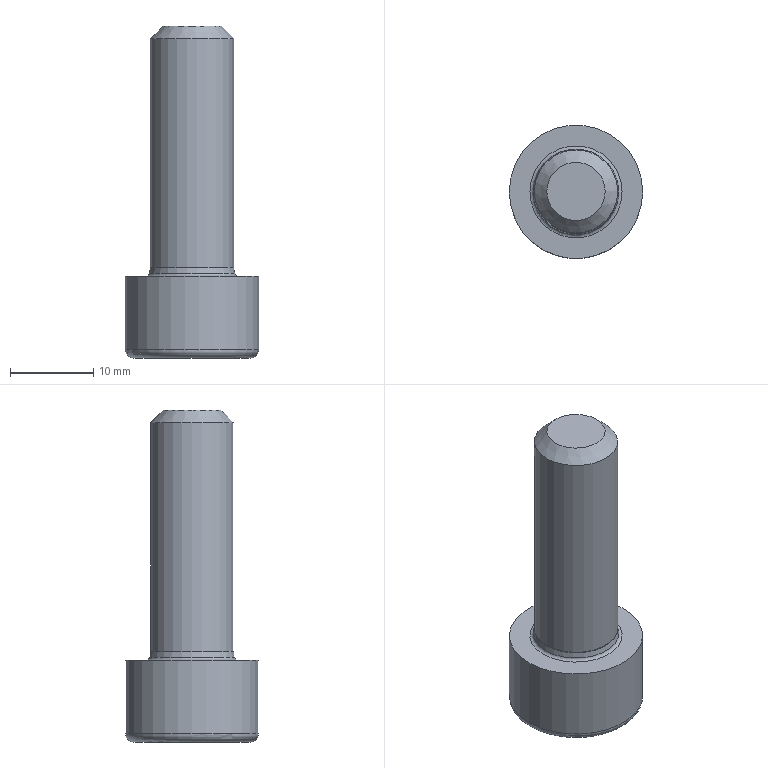Component | NX | CA6140-ZHUZHOU-LUODING | 1 solid | 17 faces | volume 4032 mm3 | plane 9 | cone 3 | torus 3 | cylinder 2 | commonest cylinder face diameters 10 x1 16 x1